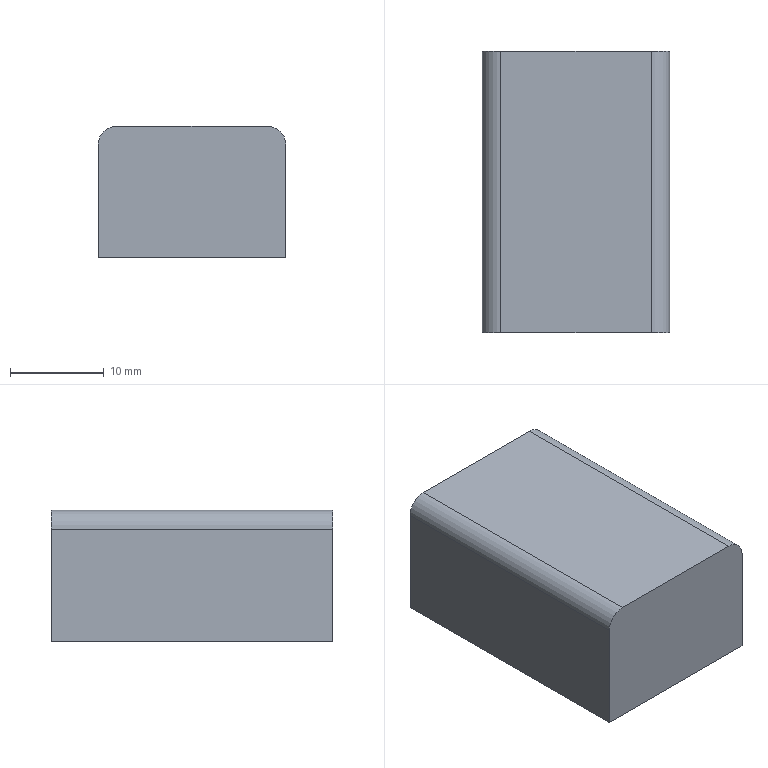Component | SolidWorks | LongSideClampingAssemblyBGeneralAssembly-1_FrictionBlockB-0510-1 | 1 solid | 12 faces | box 20 x 30 x 14 mm | volume 7984 mm3 | plane 6 | cylinder 4 | cone 2 | commonest cylinder face diameters 6.6 x2 4 x2 | material Brass
build123d program:
from build123d import *

# Parameters (mm, degrees)
SKETCH1_W                 = 30
SKETCH1_H                 = 20
BOSS_EXTRUDE1_DEPTH       = 14
M6_CLEARANCE_HOLE_1_D     = 6.6
M6_CLEARANCE_HOLE_1_DEPTH = 10
M6_CLEARANCE_HOLE_1_TIP   = 1.983
FILLET1_R                 = 2


with BuildPart() as part:
    # Sketch1 → Boss-Extrude1 (new body)
    with BuildSketch(Plane(origin=(0, 0, 0), x_dir=(0, 0, -1), z_dir=(1, 0, 0))):
        Rectangle(SKETCH1_W, SKETCH1_H)
    extrude(amount=BOSS_EXTRUDE1_DEPTH)

    # M6 Clearance Hole 1
    with Locations(Plane(origin=(14, 0, 0), x_dir=(0, 0, -1), z_dir=(1, 0, 0))):
        with Locations((0, 0)):
            Hole(M6_CLEARANCE_HOLE_1_D / 2, depth=M6_CLEARANCE_HOLE_1_DEPTH)
            with Locations((0, 0, -(M6_CLEARANCE_HOLE_1_DEPTH + M6_CLEARANCE_HOLE_1_TIP / 2))):  # 118° drill point
                Cone(0, M6_CLEARANCE_HOLE_1_D / 2, M6_CLEARANCE_HOLE_1_TIP, mode=Mode.SUBTRACT)

    # Fillet1
    fillet1_edges = [part.edges().sort_by_distance(p)[0] for p in [
        (0, -10, 0),
        (0, 10, 0),
    ]]
    fillet(fillet1_edges, radius=FILLET1_R)


solid = part.part

# Placed as in the assembly
solid = solid.moved(Location((-3230.658, 0.3914, 3515), (90, 0, -90)))
STEP:
#1=CARTESIAN_POINT('',(-127.191,-0.1145,138.228));
#2=VERTEX_POINT('',#1);
#3=CARTESIAN_POINT('',(-127.191,0.1453,138.228));
#4=VERTEX_POINT('',#3);
#5=CARTESIAN_POINT('',(-127.191,0.01541,138.228));
#6=DIRECTION('',(-0.,-0.,-1.));
#7=DIRECTION('',(0.,1.,0.));
#8=AXIS2_PLACEMENT_3D('',#5,#6,#7);
#9=CIRCLE('',#8,0.1299);
#10=EDGE_CURVE('',#2,#4,#9,.T.);
#11=ORIENTED_EDGE('',*,*,#10,.F.);
#12=CARTESIAN_POINT('',(-127.191,-0.1145,137.835));
#13=VERTEX_POINT('',#12);
#14=CARTESIAN_POINT('',(-127.191,-0.1145,137.835));
#15=DIRECTION('',(-0.,-0.,-1.));
#16=VECTOR('',#15,39.37);
#17=LINE('',#14,#16);
#18=EDGE_CURVE('',#2,#13,#17,.T.);
#19=ORIENTED_EDGE('',*,*,#18,.T.);
#20=CARTESIAN_POINT('',(-127.191,0.1453,137.835));
#21=VERTEX_POINT('',#20);
#22=CARTESIAN_POINT('',(-127.191,0.01541,137.835));
#23=DIRECTION('',(-0.,-0.,-1.));
#24=DIRECTION('',(0.,1.,0.));
#25=AXIS2_PLACEMENT_3D('',#22,#23,#24);
#26=CIRCLE('',#25,0.1299);
#27=EDGE_CURVE('',#13,#21,#26,.T.);
#28=ORIENTED_EDGE('',*,*,#27,.T.);
#29=CARTESIAN_POINT('',(-127.191,0.1453,137.835));
#30=DIRECTION('',(-0.,-0.,-1.));
#31=VECTOR('',#30,39.37);
#32=LINE('',#29,#31);
#33=EDGE_CURVE('',#4,#21,#32,.T.);
#34=ORIENTED_EDGE('',*,*,#33,.F.);
#35=EDGE_LOOP('',(#11,#19,#28,#34));
#36=FACE_OUTER_BOUND('',#35,.T.);
#37=CARTESIAN_POINT('',(-127.191,0.01541,137.835));
#38=DIRECTION('',(-0.,-0.,-1.));
#39=DIRECTION('',(0.,1.,0.));
#40=AXIS2_PLACEMENT_3D('',#37,#38,#39);
#41=CYLINDRICAL_SURFACE('',#40,0.1299);
#42=ADVANCED_FACE('',(#36),#41,.F.);
#43=CARTESIAN_POINT('',(-127.191,0.01541,138.306));
#44=VERTEX_POINT('',#43);
#45=CARTESIAN_POINT('',(-127.191,0.1453,138.228));
#46=DIRECTION('',(0.,0.8572,-0.515));
#47=VECTOR('',#46,39.37);
#48=LINE('',#45,#47);
#49=EDGE_CURVE('',#44,#4,#48,.T.);
#50=ORIENTED_EDGE('',*,*,#49,.F.);
#51=CARTESIAN_POINT('',(-127.191,-0.1145,138.228));
#52=DIRECTION('',(-0.,-0.8572,-0.515));
#53=VECTOR('',#52,39.37);
#54=LINE('',#51,#53);
#55=EDGE_CURVE('',#44,#2,#54,.T.);
#56=ORIENTED_EDGE('',*,*,#55,.T.);
#57=ORIENTED_EDGE('',*,*,#10,.T.);
#58=EDGE_LOOP('',(#50,#56,#57));
#59=FACE_OUTER_BOUND('',#58,.T.);
#60=CARTESIAN_POINT('',(-127.191,0.01541,138.228));
#61=DIRECTION('',(-0.,-0.,-1.));
#62=DIRECTION('',(0.,1.,0.));
#63=AXIS2_PLACEMENT_3D('',#60,#61,#62);
#64=CONICAL_SURFACE('',#63,0.1299,1.03);
#65=ADVANCED_FACE('',(#59),#64,.F.);
#66=CARTESIAN_POINT('',(-127.506,0.606,138.386));
#67=VERTEX_POINT('',#66);
#68=CARTESIAN_POINT('',(-126.876,0.606,138.386));
#69=VERTEX_POINT('',#68);
#70=CARTESIAN_POINT('',(-127.585,0.606,138.386));
#71=DIRECTION('',(1.,-0.,-0.));
#72=VECTOR('',#71,39.37);
#73=LINE('',#70,#72);
#74=EDGE_CURVE('',#67,#69,#73,.T.);
#75=ORIENTED_EDGE('',*,*,#74,.T.);
#76=CARTESIAN_POINT('',(-126.798,0.606,138.307));
#77=VERTEX_POINT('',#76);
#78=CARTESIAN_POINT('',(-126.876,0.606,138.307));
#79=DIRECTION('',(0.,1.,-0.));
#80=DIRECTION('',(0.,0.,-1.));
#81=AXIS2_PLACEMENT_3D('',#78,#79,#80);
#82=CIRCLE('',#81,0.07874);
#83=EDGE_CURVE('',#69,#77,#82,.T.);
#84=ORIENTED_EDGE('',*,*,#83,.T.);
#85=CARTESIAN_POINT('',(-126.798,0.606,137.835));
#86=VERTEX_POINT('',#85);
#87=CARTESIAN_POINT('',(-126.798,0.606,137.835));
#88=DIRECTION('',(0.,0.,1.));
#89=VECTOR('',#88,39.37);
#90=LINE('',#87,#89);
#91=EDGE_CURVE('',#86,#77,#90,.T.);
#92=ORIENTED_EDGE('',*,*,#91,.F.);
#93=CARTESIAN_POINT('',(-127.585,0.606,137.835));
#94=VERTEX_POINT('',#93);
#95=CARTESIAN_POINT('',(-127.585,0.606,137.835));
#96=DIRECTION('',(1.,-0.,-0.));
#97=VECTOR('',#96,39.37);
#98=LINE('',#95,#97);
#99=EDGE_CURVE('',#94,#86,#98,.T.);
#100=ORIENTED_EDGE('',*,*,#99,.F.);
#101=CARTESIAN_POINT('',(-127.585,0.606,138.307));
#102=VERTEX_POINT('',#101);
#103=CARTESIAN_POINT('',(-127.585,0.606,137.835));
#104=DIRECTION('',(0.,0.,1.));
#105=VECTOR('',#104,39.37);
#106=LINE('',#103,#105);
#107=EDGE_CURVE('',#94,#102,#106,.T.);
#108=ORIENTED_EDGE('',*,*,#107,.T.);
#109=CARTESIAN_POINT('',(-127.506,0.606,138.307));
#110=DIRECTION('',(0.,1.,-0.));
#111=DIRECTION('',(0.,0.,-1.));
#112=AXIS2_PLACEMENT_3D('',#109,#110,#111);
#113=CIRCLE('',#112,0.07874);
#114=EDGE_CURVE('',#102,#67,#113,.T.);
#115=ORIENTED_EDGE('',*,*,#114,.T.);
#116=EDGE_LOOP('',(#75,#84,#92,#100,#108,#115));
#117=FACE_OUTER_BOUND('',#116,.T.);
#118=CARTESIAN_POINT('',(-127.585,0.606,137.835));
#119=DIRECTION('',(-0.,-1.,0.));
#120=DIRECTION('',(-0.,-0.,-1.));
#121=AXIS2_PLACEMENT_3D('',#118,#119,#120);
#122=PLANE('',#121);
#123=ADVANCED_FACE('',(#117),#122,.F.);
#124=ORIENTED_EDGE('',*,*,#91,.T.);
#125=CARTESIAN_POINT('',(-126.798,-0.5751,138.307));
#126=VERTEX_POINT('',#125);
#127=CARTESIAN_POINT('',(-126.798,-0.5751,138.307));
#128=DIRECTION('',(-0.,-1.,0.));
#129=VECTOR('',#128,39.37);
#130=LINE('',#127,#129);
#131=EDGE_CURVE('',#77,#126,#130,.T.);
#132=ORIENTED_EDGE('',*,*,#131,.T.);
#133=CARTESIAN_POINT('',(-126.798,-0.5751,137.835));
#134=VERTEX_POINT('',#133);
#135=CARTESIAN_POINT('',(-126.798,-0.5751,137.835));
#136=DIRECTION('',(0.,0.,1.));
#137=VECTOR('',#136,39.37);
#138=LINE('',#135,#137);
#139=EDGE_CURVE('',#134,#126,#138,.T.);
#140=ORIENTED_EDGE('',*,*,#139,.F.);
#141=CARTESIAN_POINT('',(-126.798,-0.5751,137.835));
#142=DIRECTION('',(-0.,-1.,0.));
#143=VECTOR('',#142,39.37);
#144=LINE('',#141,#143);
#145=EDGE_CURVE('',#86,#134,#144,.T.);
#146=ORIENTED_EDGE('',*,*,#145,.F.);
#147=EDGE_LOOP('',(#124,#132,#140,#146));
#148=FACE_OUTER_BOUND('',#147,.T.);
#149=CARTESIAN_POINT('',(-126.798,-0.5751,137.835));
#150=DIRECTION('',(-1.,0.,0.));
#151=DIRECTION('',(0.,1.,-0.));
#152=AXIS2_PLACEMENT_3D('',#149,#150,#151);
#153=PLANE('',#152);
#154=ADVANCED_FACE('',(#148),#153,.F.);
#155=ORIENTED_EDGE('',*,*,#139,.T.);
#156=CARTESIAN_POINT('',(-126.876,-0.5751,138.386));
#157=VERTEX_POINT('',#156);
#158=CARTESIAN_POINT('',(-126.876,-0.5751,138.307));
#159=DIRECTION('',(-0.,-1.,0.));
#160=DIRECTION('',(0.,0.,1.));
#161=AXIS2_PLACEMENT_3D('',#158,#159,#160);
#162=CIRCLE('',#161,0.07874);
#163=EDGE_CURVE('',#126,#157,#162,.T.);
#164=ORIENTED_EDGE('',*,*,#163,.T.);
#165=CARTESIAN_POINT('',(-127.506,-0.5751,138.386));
#166=VERTEX_POINT('',#165);
#167=CARTESIAN_POINT('',(-127.585,-0.5751,138.386));
#168=DIRECTION('',(-1.,0.,0.));
#169=VECTOR('',#168,39.37);
#170=LINE('',#167,#169);
#171=EDGE_CURVE('',#157,#166,#170,.T.);
#172=ORIENTED_EDGE('',*,*,#171,.T.);
#173=CARTESIAN_POINT('',(-127.585,-0.5751,138.307));
#174=VERTEX_POINT('',#173);
#175=CARTESIAN_POINT('',(-127.506,-0.5751,138.307));
#176=DIRECTION('',(-0.,-1.,0.));
#177=DIRECTION('',(0.,0.,1.));
#178=AXIS2_PLACEMENT_3D('',#175,#176,#177);
#179=CIRCLE('',#178,0.07874);
#180=EDGE_CURVE('',#166,#174,#179,.T.);
#181=ORIENTED_EDGE('',*,*,#180,.T.);
#182=CARTESIAN_POINT('',(-127.585,-0.5751,137.835));
#183=VERTEX_POINT('',#182);
#184=CARTESIAN_POINT('',(-127.585,-0.5751,137.835));
#185=DIRECTION('',(0.,0.,1.));
#186=VECTOR('',#185,39.37);
#187=LINE('',#184,#186);
#188=EDGE_CURVE('',#183,#174,#187,.T.);
#189=ORIENTED_EDGE('',*,*,#188,.F.);
#190=CARTESIAN_POINT('',(-127.585,-0.5751,137.835));
#191=DIRECTION('',(-1.,0.,0.));
#192=VECTOR('',#191,39.37);
#193=LINE('',#190,#192);
#194=EDGE_CURVE('',#134,#183,#193,.T.);
#195=ORIENTED_EDGE('',*,*,#194,.F.);
#196=EDGE_LOOP('',(#155,#164,#172,#181,#189,#195));
#197=FACE_OUTER_BOUND('',#196,.T.);
#198=CARTESIAN_POINT('',(-127.585,-0.5751,137.835));
#199=DIRECTION('',(0.,1.,-0.));
#200=DIRECTION('',(0.,0.,1.));
#201=AXIS2_PLACEMENT_3D('',#198,#199,#200);
#202=PLANE('',#201);
#203=ADVANCED_FACE('',(#197),#202,.F.);
#204=ORIENTED_EDGE('',*,*,#188,.T.);
#205=CARTESIAN_POINT('',(-127.585,0.606,138.307));
#206=DIRECTION('',(0.,1.,-0.));
#207=VECTOR('',#206,39.37);
#208=LINE('',#205,#207);
#209=EDGE_CURVE('',#174,#102,#208,.T.);
#210=ORIENTED_EDGE('',*,*,#209,.T.);
#211=ORIENTED_EDGE('',*,*,#107,.F.);
#212=CARTESIAN_POINT('',(-127.585,-0.5751,137.835));
#213=DIRECTION('',(0.,1.,-0.));
#214=VECTOR('',#213,39.37);
#215=LINE('',#212,#214);
#216=EDGE_CURVE('',#183,#94,#215,.T.);
#217=ORIENTED_EDGE('',*,*,#216,.F.);
#218=EDGE_LOOP('',(#204,#210,#211,#217));
#219=FACE_OUTER_BOUND('',#218,.T.);
#220=CARTESIAN_POINT('',(-127.585,-0.5751,137.835));
#221=DIRECTION('',(1.,-0.,-0.));
#222=DIRECTION('',(-0.,-1.,0.));
#223=AXIS2_PLACEMENT_3D('',#220,#221,#222);
#224=PLANE('',#223);
#225=ADVANCED_FACE('',(#219),#224,.F.);
#226=CARTESIAN_POINT('',(-127.191,0.01541,137.835));
#227=DIRECTION('',(-0.,-0.,-1.));
#228=DIRECTION('',(0.,1.,0.));
#229=AXIS2_PLACEMENT_3D('',#226,#227,#228);
#230=CIRCLE('',#229,0.1299);
#231=EDGE_CURVE('',#21,#13,#230,.T.);
#232=ORIENTED_EDGE('',*,*,#231,.F.);
#233=ORIENTED_EDGE('',*,*,#27,.F.);
#234=EDGE_LOOP('',(#232,#233));
#235=FACE_BOUND('',#234,.T.);
#236=ORIENTED_EDGE('',*,*,#99,.T.);
#237=ORIENTED_EDGE('',*,*,#145,.T.);
#238=ORIENTED_EDGE('',*,*,#194,.T.);
#239=ORIENTED_EDGE('',*,*,#216,.T.);
#240=EDGE_LOOP('',(#236,#237,#238,#239));
#241=FACE_OUTER_BOUND('',#240,.T.);
#242=CARTESIAN_POINT('',(-127.191,0.01541,137.835));
#243=DIRECTION('',(0.,0.,1.));
#244=DIRECTION('',(-0.,-1.,0.));
#245=AXIS2_PLACEMENT_3D('',#242,#243,#244);
#246=PLANE('',#245);
#247=ADVANCED_FACE('',(#235,#241),#246,.F.);
#248=ORIENTED_EDGE('',*,*,#171,.F.);
#249=CARTESIAN_POINT('',(-126.876,0.606,138.386));
#250=DIRECTION('',(0.,1.,-0.));
#251=VECTOR('',#250,39.37);
#252=LINE('',#249,#251);
#253=EDGE_CURVE('',#157,#69,#252,.T.);
#254=ORIENTED_EDGE('',*,*,#253,.T.);
#255=ORIENTED_EDGE('',*,*,#74,.F.);
#256=CARTESIAN_POINT('',(-127.506,-0.5751,138.386));
#257=DIRECTION('',(-0.,-1.,0.));
#258=VECTOR('',#257,39.37);
#259=LINE('',#256,#258);
#260=EDGE_CURVE('',#67,#166,#259,.T.);
#261=ORIENTED_EDGE('',*,*,#260,.T.);
#262=EDGE_LOOP('',(#248,#254,#255,#261));
#263=FACE_OUTER_BOUND('',#262,.T.);
#264=CARTESIAN_POINT('',(-127.191,0.01541,138.386));
#265=DIRECTION('',(0.,0.,1.));
#266=DIRECTION('',(-0.,-1.,0.));
#267=AXIS2_PLACEMENT_3D('',#264,#265,#266);
#268=PLANE('',#267);
#269=ADVANCED_FACE('',(#263),#268,.T.);
#270=ORIENTED_EDGE('',*,*,#55,.F.);
#271=ORIENTED_EDGE('',*,*,#49,.T.);
#272=CARTESIAN_POINT('',(-127.191,0.01541,138.228));
#273=DIRECTION('',(-0.,-0.,-1.));
#274=DIRECTION('',(0.,1.,0.));
#275=AXIS2_PLACEMENT_3D('',#272,#273,#274);
#276=CIRCLE('',#275,0.1299);
#277=EDGE_CURVE('',#4,#2,#276,.T.);
#278=ORIENTED_EDGE('',*,*,#277,.T.);
#279=EDGE_LOOP('',(#270,#271,#278));
#280=FACE_OUTER_BOUND('',#279,.T.);
#281=CARTESIAN_POINT('',(-127.191,0.01541,138.228));
#282=DIRECTION('',(-0.,-0.,-1.));
#283=DIRECTION('',(0.,1.,0.));
#284=AXIS2_PLACEMENT_3D('',#281,#282,#283);
#285=CONICAL_SURFACE('',#284,0.1299,1.03);
#286=ADVANCED_FACE('',(#280),#285,.F.);
#287=ORIENTED_EDGE('',*,*,#18,.F.);
#288=ORIENTED_EDGE('',*,*,#277,.F.);
#289=ORIENTED_EDGE('',*,*,#33,.T.);
#290=ORIENTED_EDGE('',*,*,#231,.T.);
#291=EDGE_LOOP('',(#287,#288,#289,#290));
#292=FACE_OUTER_BOUND('',#291,.T.);
#293=CARTESIAN_POINT('',(-127.191,0.01541,137.835));
#294=DIRECTION('',(-0.,-0.,-1.));
#295=DIRECTION('',(0.,1.,0.));
#296=AXIS2_PLACEMENT_3D('',#293,#294,#295);
#297=CYLINDRICAL_SURFACE('',#296,0.1299);
#298=ADVANCED_FACE('',(#292),#297,.F.);
#299=ORIENTED_EDGE('',*,*,#83,.F.);
#300=ORIENTED_EDGE('',*,*,#253,.F.);
#301=ORIENTED_EDGE('',*,*,#163,.F.);
#302=ORIENTED_EDGE('',*,*,#131,.F.);
#303=EDGE_LOOP('',(#299,#300,#301,#302));
#304=FACE_OUTER_BOUND('',#303,.T.);
#305=CARTESIAN_POINT('',(-126.876,-0.5751,138.307));
#306=DIRECTION('',(0.,1.,-0.));
#307=DIRECTION('',(0.,0.,1.));
#308=AXIS2_PLACEMENT_3D('',#305,#306,#307);
#309=CYLINDRICAL_SURFACE('',#308,0.07874);
#310=ADVANCED_FACE('',(#304),#309,.T.);
#311=ORIENTED_EDGE('',*,*,#180,.F.);
#312=ORIENTED_EDGE('',*,*,#260,.F.);
#313=ORIENTED_EDGE('',*,*,#114,.F.);
#314=ORIENTED_EDGE('',*,*,#209,.F.);
#315=EDGE_LOOP('',(#311,#312,#313,#314));
#316=FACE_OUTER_BOUND('',#315,.T.);
#317=CARTESIAN_POINT('',(-127.506,-0.5751,138.307));
#318=DIRECTION('',(-0.,-1.,0.));
#319=DIRECTION('',(0.,0.,-1.));
#320=AXIS2_PLACEMENT_3D('',#317,#318,#319);
#321=CYLINDRICAL_SURFACE('',#320,0.07874);
#322=ADVANCED_FACE('',(#316),#321,.T.);
#323=CLOSED_SHELL('',(#42,#65,#123,#154,#203,#225,#247,#269,#286,#298,#310,#322));
#324=MANIFOLD_SOLID_BREP('',#323);
#325=CARTESIAN_POINT('',(0.,0.,0.));
#326=DIRECTION('',(0.,0.,1.));
#327=DIRECTION('',(1.,0.,0.));
#328=AXIS2_PLACEMENT_3D('',#325,#326,#327);
#329=(LENGTH_UNIT()NAMED_UNIT(*)SI_UNIT($,.METRE.));
#330=LENGTH_MEASURE_WITH_UNIT(LENGTH_MEASURE(0.0254),#329);
#331=DIMENSIONAL_EXPONENTS(1.,0.,0.,0.,0.,0.,0.);
#332=(CONVERSION_BASED_UNIT('',#330)LENGTH_UNIT()NAMED_UNIT(#331));
#333=UNCERTAINTY_MEASURE_WITH_UNIT(LENGTH_MEASURE(0.00001),#332,'','');
#334=(NAMED_UNIT(*)PLANE_ANGLE_UNIT()SI_UNIT($,.RADIAN.));
#335=(NAMED_UNIT(*)SI_UNIT($,.STERADIAN.)SOLID_ANGLE_UNIT());
#336=(GEOMETRIC_REPRESENTATION_CONTEXT(3)GLOBAL_UNCERTAINTY_ASSIGNED_CONTEXT((#333))GLOBAL_UNIT_ASSIGNED_CONTEXT((#332,#334,#335))REPRESENTATION_CONTEXT('',''));
#337=ADVANCED_BREP_SHAPE_REPRESENTATION('',(#324,#328),#336);
#338=COLOUR_RGB('',0.7922,0.8196,0.9333);
#339=FILL_AREA_STYLE_COLOUR('',#338);
#340=FILL_AREA_STYLE('',(#339));
#341=SURFACE_STYLE_FILL_AREA(#340);
#342=SURFACE_SIDE_STYLE('',(#341));
#343=SURFACE_STYLE_USAGE(.BOTH.,#342);
#344=PRESENTATION_STYLE_ASSIGNMENT((#343));
#345=STYLED_ITEM('',(#344),#324);
#346=PRESENTATION_LAYER_ASSIGNMENT('','',(#345));
#347=(LENGTH_UNIT()NAMED_UNIT(*)SI_UNIT($,.METRE.));
#348=LENGTH_MEASURE_WITH_UNIT(LENGTH_MEASURE(0.0254),#347);
#349=DIMENSIONAL_EXPONENTS(1.,0.,0.,0.,0.,0.,0.);
#350=(CONVERSION_BASED_UNIT('',#348)LENGTH_UNIT()NAMED_UNIT(#349));
#351=UNCERTAINTY_MEASURE_WITH_UNIT(LENGTH_MEASURE(0.00001),#350,'','');
#352=(NAMED_UNIT(*)PLANE_ANGLE_UNIT()SI_UNIT($,.RADIAN.));
#353=(NAMED_UNIT(*)SI_UNIT($,.STERADIAN.)SOLID_ANGLE_UNIT());
#354=(GEOMETRIC_REPRESENTATION_CONTEXT(3)GLOBAL_UNCERTAINTY_ASSIGNED_CONTEXT((#351))GLOBAL_UNIT_ASSIGNED_CONTEXT((#350,#352,#353))REPRESENTATION_CONTEXT('',''));
#355=MECHANICAL_DESIGN_GEOMETRIC_PRESENTATION_REPRESENTATION('',(#345),#354);